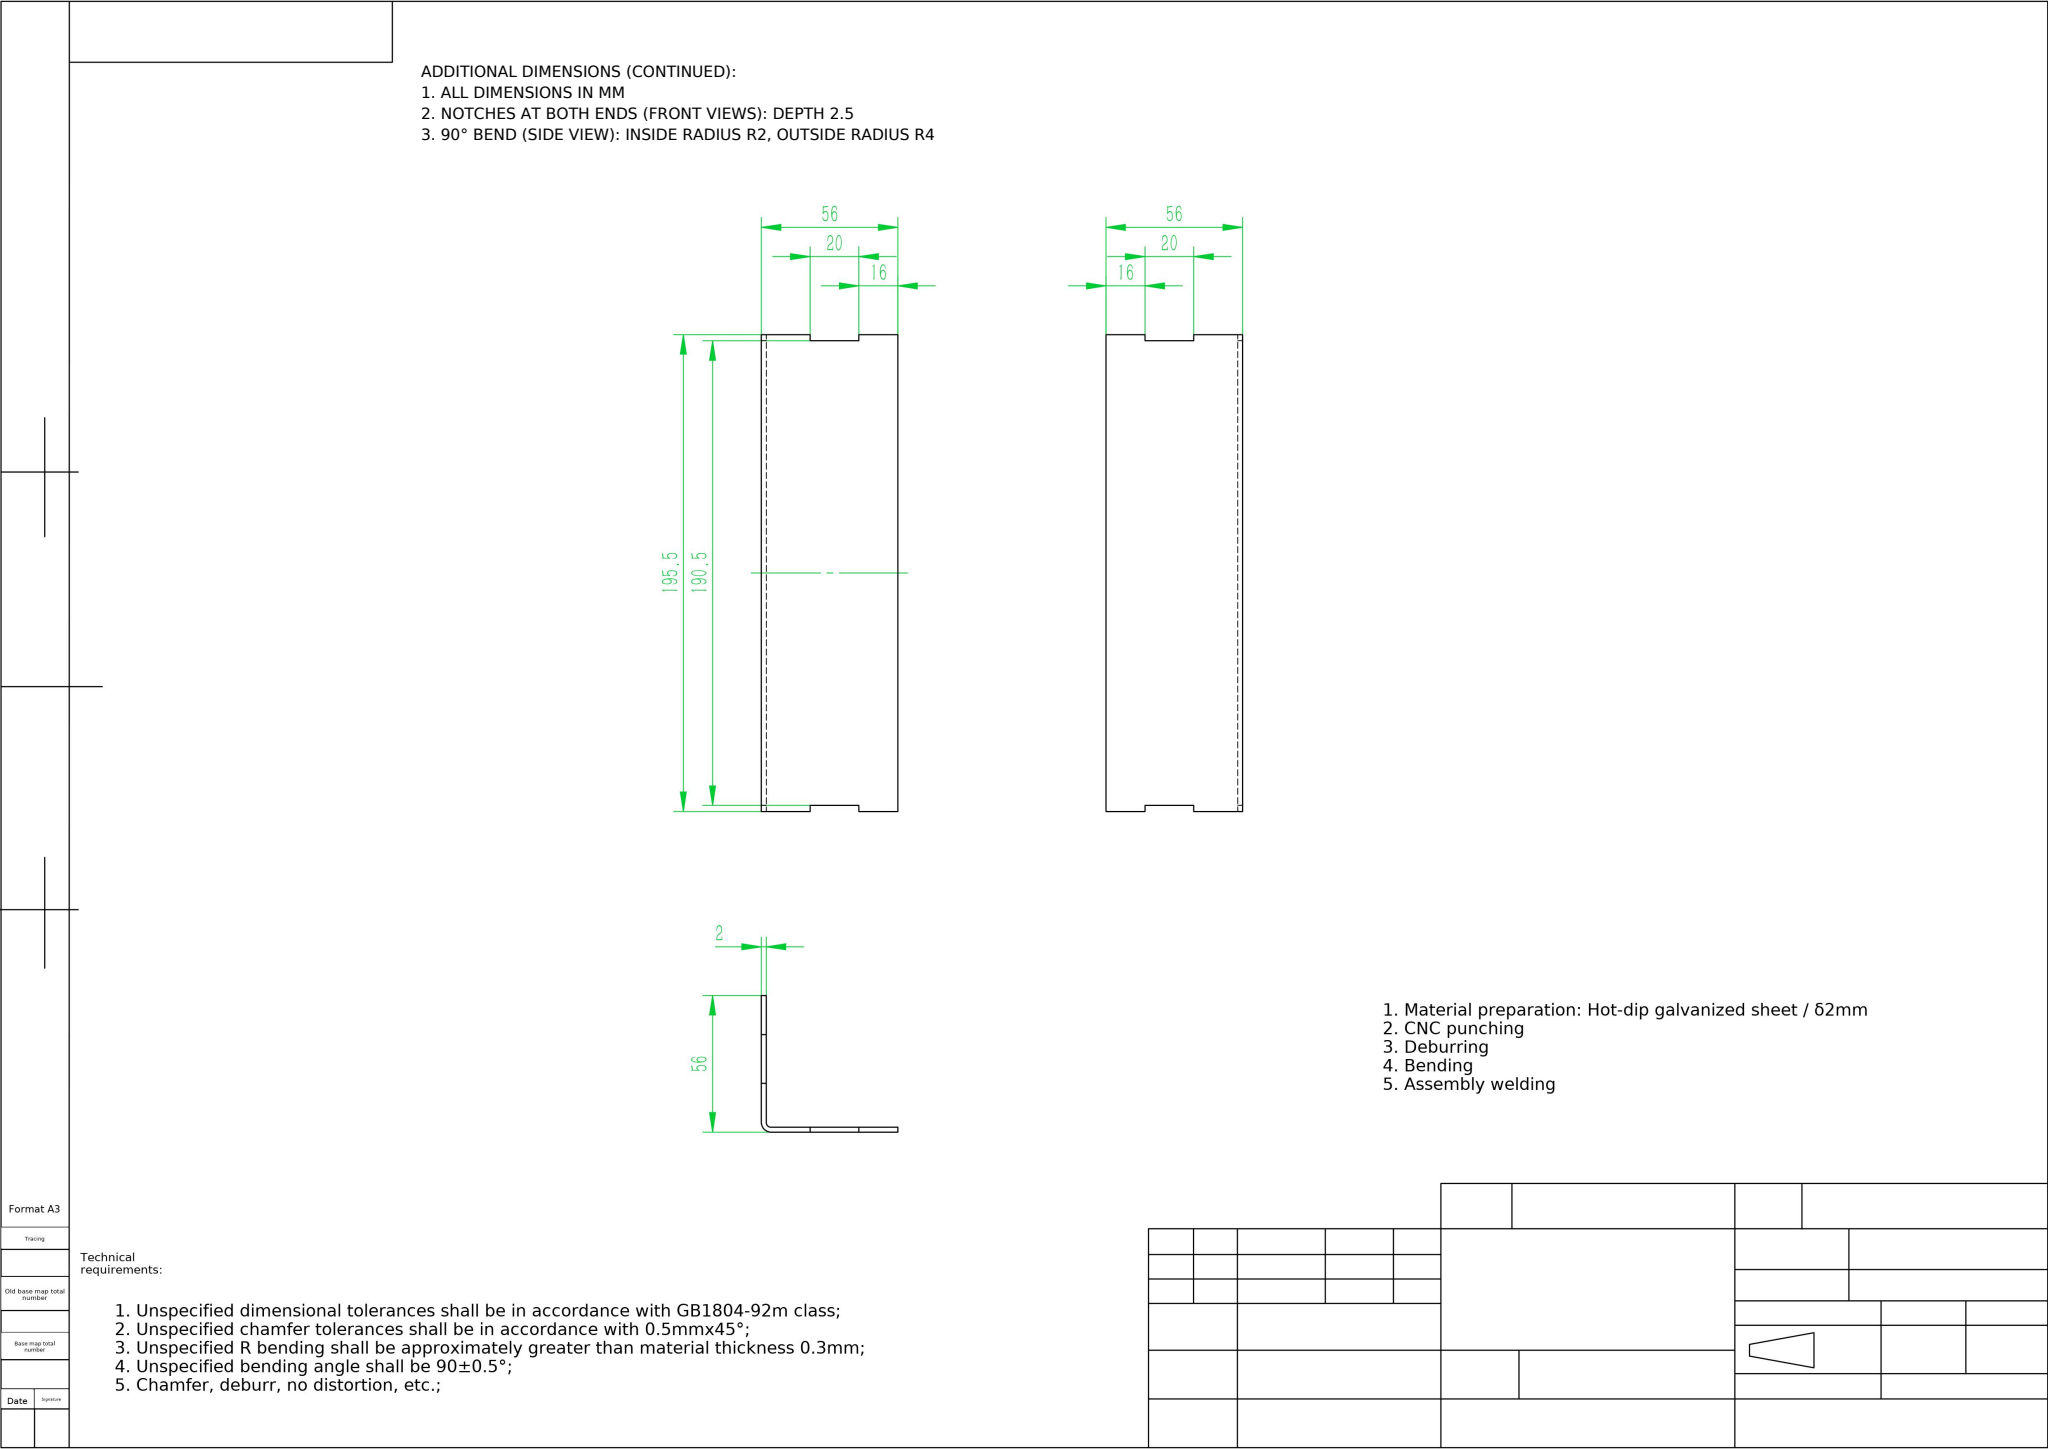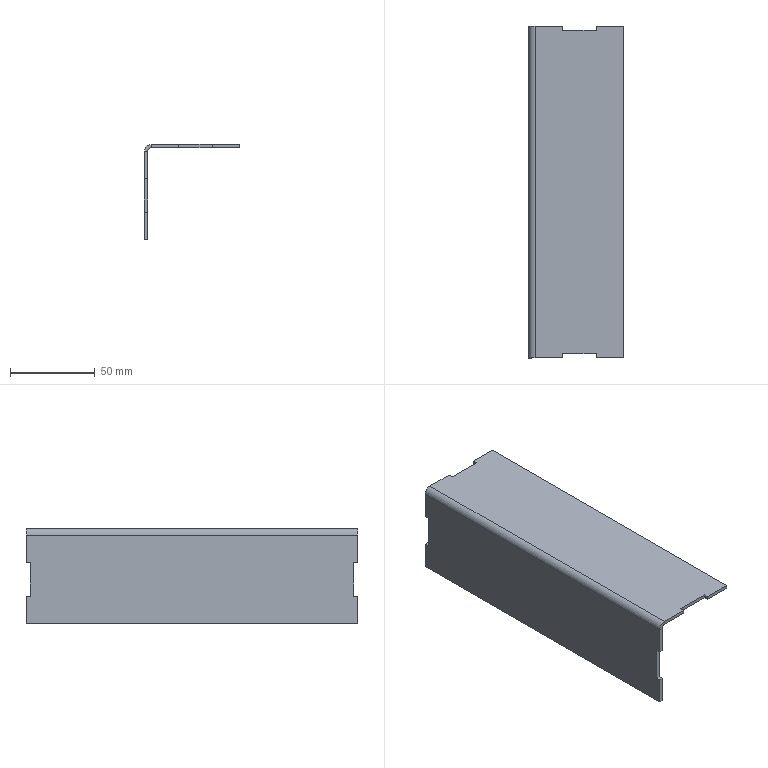Part | NX | mm | 1 solid | 30 faces | box 56 x 195.5 x 56 mm | volume 42107 mm3 | plane 28 | cylinder 2 | commonest cylinder face diameters 8 x1 4 x1
STEP:
#1=COLOUR_RGB('',0.7529,0.7529,0.7529);
#2=FILL_AREA_STYLE_COLOUR('',#1);
#3=FILL_AREA_STYLE('',(#2));
#4=SURFACE_STYLE_FILL_AREA(#3);
#5=SURFACE_SIDE_STYLE('',(#4));
#6=SURFACE_STYLE_USAGE(.BOTH.,#5);
#7=PRESENTATION_STYLE_ASSIGNMENT((#6));
#8=CARTESIAN_POINT('',(-28.,-97.75,-4.));
#9=VERTEX_POINT('',#8);
#10=CARTESIAN_POINT('',(-28.,-97.75,-20.));
#11=VERTEX_POINT('',#10);
#12=CARTESIAN_POINT('',(-28.,-97.75,-56.));
#13=DIRECTION('',(-0.,0.,-1.));
#14=VECTOR('',#13,1000.);
#15=LINE('',#12,#14);
#16=EDGE_CURVE('',#9,#11,#15,.T.);
#17=ORIENTED_EDGE('',*,*,#16,.T.);
#18=CARTESIAN_POINT('',(-26.,-97.75,-20.));
#19=VERTEX_POINT('',#18);
#20=CARTESIAN_POINT('',(-28.,-97.75,-20.));
#21=DIRECTION('',(1.,0.,-0.));
#22=VECTOR('',#21,1000.);
#23=LINE('',#20,#22);
#24=EDGE_CURVE('',#11,#19,#23,.T.);
#25=ORIENTED_EDGE('',*,*,#24,.T.);
#26=CARTESIAN_POINT('',(-26.,-97.75,-4.));
#27=VERTEX_POINT('',#26);
#28=CARTESIAN_POINT('',(-26.,-97.75,0.));
#29=DIRECTION('',(-0.,0.,-1.));
#30=VECTOR('',#29,1000.);
#31=LINE('',#28,#30);
#32=EDGE_CURVE('',#27,#19,#31,.T.);
#33=ORIENTED_EDGE('',*,*,#32,.F.);
#34=CARTESIAN_POINT('',(-28.,-97.75,-4.));
#35=DIRECTION('',(-1.,0.,0.));
#36=VECTOR('',#35,1000.);
#37=LINE('',#34,#36);
#38=EDGE_CURVE('',#27,#9,#37,.T.);
#39=ORIENTED_EDGE('',*,*,#38,.T.);
#40=EDGE_LOOP('',(#17,#25,#33,#39));
#41=FACE_OUTER_BOUND('',#40,.T.);
#42=CARTESIAN_POINT('',(-28.,-97.75,-56.));
#43=DIRECTION('',(0.,-1.,0.));
#44=DIRECTION('',(0.,0.,-1.));
#45=AXIS2_PLACEMENT_3D('',#42,#43,#44);
#46=PLANE('',#45);
#47=ADVANCED_FACE('',(#41),#46,.T.);
#48=CARTESIAN_POINT('',(-26.,-97.75,-40.));
#49=VERTEX_POINT('',#48);
#50=CARTESIAN_POINT('',(-26.,-97.75,-56.));
#51=VERTEX_POINT('',#50);
#52=CARTESIAN_POINT('',(-26.,-97.75,0.));
#53=DIRECTION('',(-0.,0.,-1.));
#54=VECTOR('',#53,1000.);
#55=LINE('',#52,#54);
#56=EDGE_CURVE('',#49,#51,#55,.T.);
#57=ORIENTED_EDGE('',*,*,#56,.F.);
#58=CARTESIAN_POINT('',(-28.,-97.75,-40.));
#59=VERTEX_POINT('',#58);
#60=CARTESIAN_POINT('',(-28.,-97.75,-40.));
#61=DIRECTION('',(-1.,0.,0.));
#62=VECTOR('',#61,1000.);
#63=LINE('',#60,#62);
#64=EDGE_CURVE('',#49,#59,#63,.T.);
#65=ORIENTED_EDGE('',*,*,#64,.T.);
#66=CARTESIAN_POINT('',(-28.,-97.75,-56.));
#67=VERTEX_POINT('',#66);
#68=CARTESIAN_POINT('',(-28.,-97.75,-56.));
#69=DIRECTION('',(-0.,0.,-1.));
#70=VECTOR('',#69,1000.);
#71=LINE('',#68,#70);
#72=EDGE_CURVE('',#59,#67,#71,.T.);
#73=ORIENTED_EDGE('',*,*,#72,.T.);
#74=CARTESIAN_POINT('',(-28.,-97.75,-56.));
#75=DIRECTION('',(1.,0.,-0.));
#76=VECTOR('',#75,1000.);
#77=LINE('',#74,#76);
#78=EDGE_CURVE('',#67,#51,#77,.T.);
#79=ORIENTED_EDGE('',*,*,#78,.T.);
#80=EDGE_LOOP('',(#57,#65,#73,#79));
#81=FACE_OUTER_BOUND('',#80,.T.);
#82=CARTESIAN_POINT('',(-28.,-97.75,-56.));
#83=DIRECTION('',(0.,-1.,0.));
#84=DIRECTION('',(0.,0.,-1.));
#85=AXIS2_PLACEMENT_3D('',#82,#83,#84);
#86=PLANE('',#85);
#87=ADVANCED_FACE('',(#81),#86,.T.);
#88=CARTESIAN_POINT('',(-28.,-95.25,-40.));
#89=VERTEX_POINT('',#88);
#90=CARTESIAN_POINT('',(-28.,-95.25,-20.));
#91=VERTEX_POINT('',#90);
#92=CARTESIAN_POINT('',(-28.,-95.25,-40.));
#93=DIRECTION('',(0.,0.,1.));
#94=VECTOR('',#93,1000.);
#95=LINE('',#92,#94);
#96=EDGE_CURVE('',#89,#91,#95,.T.);
#97=ORIENTED_EDGE('',*,*,#96,.T.);
#98=CARTESIAN_POINT('',(-28.,-100.25,-20.));
#99=DIRECTION('',(0.,-1.,0.));
#100=VECTOR('',#99,1000.);
#101=LINE('',#98,#100);
#102=EDGE_CURVE('',#91,#11,#101,.T.);
#103=ORIENTED_EDGE('',*,*,#102,.T.);
#104=ORIENTED_EDGE('',*,*,#16,.F.);
#105=CARTESIAN_POINT('',(-28.,97.75,-4.));
#106=VERTEX_POINT('',#105);
#107=CARTESIAN_POINT('',(-28.,0.,-4.));
#108=DIRECTION('',(0.,1.,0.));
#109=VECTOR('',#108,1000.);
#110=LINE('',#107,#109);
#111=EDGE_CURVE('',#9,#106,#110,.T.);
#112=ORIENTED_EDGE('',*,*,#111,.T.);
#113=CARTESIAN_POINT('',(-28.,97.75,-20.));
#114=VERTEX_POINT('',#113);
#115=CARTESIAN_POINT('',(-28.,97.75,-2.));
#116=DIRECTION('',(0.,0.,1.));
#117=VECTOR('',#116,1000.);
#118=LINE('',#115,#117);
#119=EDGE_CURVE('',#114,#106,#118,.T.);
#120=ORIENTED_EDGE('',*,*,#119,.F.);
#121=CARTESIAN_POINT('',(-28.,95.25,-20.));
#122=VERTEX_POINT('',#121);
#123=CARTESIAN_POINT('',(-28.,100.25,-20.));
#124=DIRECTION('',(0.,1.,0.));
#125=VECTOR('',#124,1000.);
#126=LINE('',#123,#125);
#127=EDGE_CURVE('',#122,#114,#126,.T.);
#128=ORIENTED_EDGE('',*,*,#127,.F.);
#129=CARTESIAN_POINT('',(-28.,95.25,-40.));
#130=VERTEX_POINT('',#129);
#131=CARTESIAN_POINT('',(-28.,95.25,-40.));
#132=DIRECTION('',(0.,0.,1.));
#133=VECTOR('',#132,1000.);
#134=LINE('',#131,#133);
#135=EDGE_CURVE('',#130,#122,#134,.T.);
#136=ORIENTED_EDGE('',*,*,#135,.F.);
#137=CARTESIAN_POINT('',(-28.,97.75,-40.));
#138=VERTEX_POINT('',#137);
#139=CARTESIAN_POINT('',(-28.,100.25,-40.));
#140=DIRECTION('',(0.,-1.,0.));
#141=VECTOR('',#140,1000.);
#142=LINE('',#139,#141);
#143=EDGE_CURVE('',#138,#130,#142,.T.);
#144=ORIENTED_EDGE('',*,*,#143,.F.);
#145=CARTESIAN_POINT('',(-28.,97.75,-56.));
#146=VERTEX_POINT('',#145);
#147=CARTESIAN_POINT('',(-28.,97.75,-2.));
#148=DIRECTION('',(0.,0.,1.));
#149=VECTOR('',#148,1000.);
#150=LINE('',#147,#149);
#151=EDGE_CURVE('',#146,#138,#150,.T.);
#152=ORIENTED_EDGE('',*,*,#151,.F.);
#153=CARTESIAN_POINT('',(-28.,97.75,-56.));
#154=DIRECTION('',(0.,1.,0.));
#155=VECTOR('',#154,1000.);
#156=LINE('',#153,#155);
#157=EDGE_CURVE('',#67,#146,#156,.T.);
#158=ORIENTED_EDGE('',*,*,#157,.F.);
#159=ORIENTED_EDGE('',*,*,#72,.F.);
#160=CARTESIAN_POINT('',(-28.,-100.25,-40.));
#161=DIRECTION('',(0.,1.,0.));
#162=VECTOR('',#161,1000.);
#163=LINE('',#160,#162);
#164=EDGE_CURVE('',#59,#89,#163,.T.);
#165=ORIENTED_EDGE('',*,*,#164,.T.);
#166=EDGE_LOOP('',(#97,#103,#104,#112,#120,#128,#136,#144,#152,#158,#159,#165));
#167=FACE_OUTER_BOUND('',#166,.T.);
#168=CARTESIAN_POINT('',(-28.,0.,0.));
#169=DIRECTION('',(-1.,0.,0.));
#170=DIRECTION('',(0.,0.,1.));
#171=AXIS2_PLACEMENT_3D('',#168,#169,#170);
#172=PLANE('',#171);
#173=ADVANCED_FACE('',(#167),#172,.T.);
#174=CARTESIAN_POINT('',(-26.,-95.25,-20.));
#175=VERTEX_POINT('',#174);
#176=CARTESIAN_POINT('',(-26.,-100.25,-20.));
#177=DIRECTION('',(0.,-1.,0.));
#178=VECTOR('',#177,1000.);
#179=LINE('',#176,#178);
#180=EDGE_CURVE('',#175,#19,#179,.T.);
#181=ORIENTED_EDGE('',*,*,#180,.F.);
#182=CARTESIAN_POINT('',(-26.,-95.25,-40.));
#183=VERTEX_POINT('',#182);
#184=CARTESIAN_POINT('',(-26.,-95.25,-40.));
#185=DIRECTION('',(0.,0.,1.));
#186=VECTOR('',#185,1000.);
#187=LINE('',#184,#186);
#188=EDGE_CURVE('',#183,#175,#187,.T.);
#189=ORIENTED_EDGE('',*,*,#188,.F.);
#190=CARTESIAN_POINT('',(-26.,0.,-40.));
#191=DIRECTION('',(0.,1.,0.));
#192=VECTOR('',#191,1000.);
#193=LINE('',#190,#192);
#194=EDGE_CURVE('',#49,#183,#193,.T.);
#195=ORIENTED_EDGE('',*,*,#194,.F.);
#196=ORIENTED_EDGE('',*,*,#56,.T.);
#197=CARTESIAN_POINT('',(-26.,97.75,-56.));
#198=VERTEX_POINT('',#197);
#199=CARTESIAN_POINT('',(-26.,0.,-56.));
#200=DIRECTION('',(0.,1.,0.));
#201=VECTOR('',#200,1000.);
#202=LINE('',#199,#201);
#203=EDGE_CURVE('',#51,#198,#202,.T.);
#204=ORIENTED_EDGE('',*,*,#203,.T.);
#205=CARTESIAN_POINT('',(-26.,97.75,-40.));
#206=VERTEX_POINT('',#205);
#207=CARTESIAN_POINT('',(-26.,97.75,0.));
#208=DIRECTION('',(0.,0.,1.));
#209=VECTOR('',#208,1000.);
#210=LINE('',#207,#209);
#211=EDGE_CURVE('',#198,#206,#210,.T.);
#212=ORIENTED_EDGE('',*,*,#211,.T.);
#213=CARTESIAN_POINT('',(-26.,95.25,-40.));
#214=VERTEX_POINT('',#213);
#215=CARTESIAN_POINT('',(-26.,0.,-40.));
#216=DIRECTION('',(0.,-1.,0.));
#217=VECTOR('',#216,1000.);
#218=LINE('',#215,#217);
#219=EDGE_CURVE('',#206,#214,#218,.T.);
#220=ORIENTED_EDGE('',*,*,#219,.T.);
#221=CARTESIAN_POINT('',(-26.,95.25,-20.));
#222=VERTEX_POINT('',#221);
#223=CARTESIAN_POINT('',(-26.,95.25,-40.));
#224=DIRECTION('',(0.,0.,1.));
#225=VECTOR('',#224,1000.);
#226=LINE('',#223,#225);
#227=EDGE_CURVE('',#214,#222,#226,.T.);
#228=ORIENTED_EDGE('',*,*,#227,.T.);
#229=CARTESIAN_POINT('',(-26.,97.75,-20.));
#230=VERTEX_POINT('',#229);
#231=CARTESIAN_POINT('',(-26.,100.25,-20.));
#232=DIRECTION('',(0.,1.,0.));
#233=VECTOR('',#232,1000.);
#234=LINE('',#231,#233);
#235=EDGE_CURVE('',#222,#230,#234,.T.);
#236=ORIENTED_EDGE('',*,*,#235,.T.);
#237=CARTESIAN_POINT('',(-26.,97.75,-4.));
#238=VERTEX_POINT('',#237);
#239=CARTESIAN_POINT('',(-26.,97.75,0.));
#240=DIRECTION('',(0.,0.,1.));
#241=VECTOR('',#240,1000.);
#242=LINE('',#239,#241);
#243=EDGE_CURVE('',#230,#238,#242,.T.);
#244=ORIENTED_EDGE('',*,*,#243,.T.);
#245=CARTESIAN_POINT('',(-26.,-97.75,-4.));
#246=DIRECTION('',(0.,1.,0.));
#247=VECTOR('',#246,1000.);
#248=LINE('',#245,#247);
#249=EDGE_CURVE('',#27,#238,#248,.T.);
#250=ORIENTED_EDGE('',*,*,#249,.F.);
#251=ORIENTED_EDGE('',*,*,#32,.T.);
#252=EDGE_LOOP('',(#181,#189,#195,#196,#204,#212,#220,#228,#236,#244,#250,#251));
#253=FACE_OUTER_BOUND('',#252,.T.);
#254=CARTESIAN_POINT('',(-26.,0.,0.));
#255=DIRECTION('',(-1.,0.,0.));
#256=DIRECTION('',(0.,0.,1.));
#257=AXIS2_PLACEMENT_3D('',#254,#255,#256);
#258=PLANE('',#257);
#259=ADVANCED_FACE('',(#253),#258,.F.);
#260=CARTESIAN_POINT('',(12.,-97.75,-2.));
#261=VERTEX_POINT('',#260);
#262=CARTESIAN_POINT('',(28.,-97.75,-2.));
#263=VERTEX_POINT('',#262);
#264=CARTESIAN_POINT('',(-28.,-97.75,-2.));
#265=DIRECTION('',(1.,0.,0.));
#266=VECTOR('',#265,1000.);
#267=LINE('',#264,#266);
#268=EDGE_CURVE('',#261,#263,#267,.T.);
#269=ORIENTED_EDGE('',*,*,#268,.F.);
#270=CARTESIAN_POINT('',(12.,-95.25,-2.));
#271=VERTEX_POINT('',#270);
#272=CARTESIAN_POINT('',(12.,-100.25,-2.));
#273=DIRECTION('',(0.,-1.,0.));
#274=VECTOR('',#273,1000.);
#275=LINE('',#272,#274);
#276=EDGE_CURVE('',#271,#261,#275,.T.);
#277=ORIENTED_EDGE('',*,*,#276,.F.);
#278=CARTESIAN_POINT('',(-8.,-95.25,-2.));
#279=VERTEX_POINT('',#278);
#280=CARTESIAN_POINT('',(-8.,-95.25,-2.));
#281=DIRECTION('',(1.,0.,0.));
#282=VECTOR('',#281,1000.);
#283=LINE('',#280,#282);
#284=EDGE_CURVE('',#279,#271,#283,.T.);
#285=ORIENTED_EDGE('',*,*,#284,.F.);
#286=CARTESIAN_POINT('',(-8.,-97.75,-2.));
#287=VERTEX_POINT('',#286);
#288=CARTESIAN_POINT('',(-8.,-100.25,-2.));
#289=DIRECTION('',(0.,1.,0.));
#290=VECTOR('',#289,1000.);
#291=LINE('',#288,#290);
#292=EDGE_CURVE('',#287,#279,#291,.T.);
#293=ORIENTED_EDGE('',*,*,#292,.F.);
#294=CARTESIAN_POINT('',(-24.,-97.75,-2.));
#295=VERTEX_POINT('',#294);
#296=CARTESIAN_POINT('',(-28.,-97.75,-2.));
#297=DIRECTION('',(1.,0.,0.));
#298=VECTOR('',#297,1000.);
#299=LINE('',#296,#298);
#300=EDGE_CURVE('',#295,#287,#299,.T.);
#301=ORIENTED_EDGE('',*,*,#300,.F.);
#302=CARTESIAN_POINT('',(-24.,97.75,-2.));
#303=VERTEX_POINT('',#302);
#304=CARTESIAN_POINT('',(-24.,97.75,-2.));
#305=DIRECTION('',(0.,-1.,0.));
#306=VECTOR('',#305,1000.);
#307=LINE('',#304,#306);
#308=EDGE_CURVE('',#303,#295,#307,.T.);
#309=ORIENTED_EDGE('',*,*,#308,.F.);
#310=CARTESIAN_POINT('',(-8.,97.75,-2.));
#311=VERTEX_POINT('',#310);
#312=CARTESIAN_POINT('',(-28.,97.75,-2.));
#313=DIRECTION('',(-1.,0.,0.));
#314=VECTOR('',#313,1000.);
#315=LINE('',#312,#314);
#316=EDGE_CURVE('',#311,#303,#315,.T.);
#317=ORIENTED_EDGE('',*,*,#316,.F.);
#318=CARTESIAN_POINT('',(-8.,95.25,-2.));
#319=VERTEX_POINT('',#318);
#320=CARTESIAN_POINT('',(-8.,100.25,-2.));
#321=DIRECTION('',(0.,-1.,0.));
#322=VECTOR('',#321,1000.);
#323=LINE('',#320,#322);
#324=EDGE_CURVE('',#311,#319,#323,.T.);
#325=ORIENTED_EDGE('',*,*,#324,.T.);
#326=CARTESIAN_POINT('',(12.,95.25,-2.));
#327=VERTEX_POINT('',#326);
#328=CARTESIAN_POINT('',(-8.,95.25,-2.));
#329=DIRECTION('',(1.,0.,0.));
#330=VECTOR('',#329,1000.);
#331=LINE('',#328,#330);
#332=EDGE_CURVE('',#319,#327,#331,.T.);
#333=ORIENTED_EDGE('',*,*,#332,.T.);
#334=CARTESIAN_POINT('',(12.,97.75,-2.));
#335=VERTEX_POINT('',#334);
#336=CARTESIAN_POINT('',(12.,100.25,-2.));
#337=DIRECTION('',(0.,1.,0.));
#338=VECTOR('',#337,1000.);
#339=LINE('',#336,#338);
#340=EDGE_CURVE('',#327,#335,#339,.T.);
#341=ORIENTED_EDGE('',*,*,#340,.T.);
#342=CARTESIAN_POINT('',(28.,97.75,-2.));
#343=VERTEX_POINT('',#342);
#344=CARTESIAN_POINT('',(-28.,97.75,-2.));
#345=DIRECTION('',(-1.,0.,0.));
#346=VECTOR('',#345,1000.);
#347=LINE('',#344,#346);
#348=EDGE_CURVE('',#343,#335,#347,.T.);
#349=ORIENTED_EDGE('',*,*,#348,.F.);
#350=CARTESIAN_POINT('',(28.,-97.75,-2.));
#351=DIRECTION('',(0.,1.,0.));
#352=VECTOR('',#351,1000.);
#353=LINE('',#350,#352);
#354=EDGE_CURVE('',#263,#343,#353,.T.);
#355=ORIENTED_EDGE('',*,*,#354,.F.);
#356=EDGE_LOOP('',(#269,#277,#285,#293,#301,#309,#317,#325,#333,#341,#349,#355));
#357=FACE_OUTER_BOUND('',#356,.T.);
#358=CARTESIAN_POINT('',(0.,0.,-2.));
#359=DIRECTION('',(0.,0.,-1.));
#360=DIRECTION('',(-1.,0.,0.));
#361=AXIS2_PLACEMENT_3D('',#358,#359,#360);
#362=PLANE('',#361);
#363=ADVANCED_FACE('',(#357),#362,.T.);
#364=CARTESIAN_POINT('',(12.,-95.25,0.));
#365=VERTEX_POINT('',#364);
#366=CARTESIAN_POINT('',(12.,-97.75,0.));
#367=VERTEX_POINT('',#366);
#368=CARTESIAN_POINT('',(12.,-100.25,0.));
#369=DIRECTION('',(0.,-1.,0.));
#370=VECTOR('',#369,1000.);
#371=LINE('',#368,#370);
#372=EDGE_CURVE('',#365,#367,#371,.T.);
#373=ORIENTED_EDGE('',*,*,#372,.T.);
#374=CARTESIAN_POINT('',(28.,-97.75,0.));
#375=VERTEX_POINT('',#374);
#376=CARTESIAN_POINT('',(-28.,-97.75,0.));
#377=DIRECTION('',(1.,0.,0.));
#378=VECTOR('',#377,1000.);
#379=LINE('',#376,#378);
#380=EDGE_CURVE('',#367,#375,#379,.T.);
#381=ORIENTED_EDGE('',*,*,#380,.T.);
#382=CARTESIAN_POINT('',(28.,97.75,0.));
#383=VERTEX_POINT('',#382);
#384=CARTESIAN_POINT('',(28.,-97.75,0.));
#385=DIRECTION('',(0.,1.,0.));
#386=VECTOR('',#385,1000.);
#387=LINE('',#384,#386);
#388=EDGE_CURVE('',#375,#383,#387,.T.);
#389=ORIENTED_EDGE('',*,*,#388,.T.);
#390=CARTESIAN_POINT('',(12.,97.75,0.));
#391=VERTEX_POINT('',#390);
#392=CARTESIAN_POINT('',(-28.,97.75,0.));
#393=DIRECTION('',(-1.,0.,0.));
#394=VECTOR('',#393,1000.);
#395=LINE('',#392,#394);
#396=EDGE_CURVE('',#383,#391,#395,.T.);
#397=ORIENTED_EDGE('',*,*,#396,.T.);
#398=CARTESIAN_POINT('',(12.,95.25,0.));
#399=VERTEX_POINT('',#398);
#400=CARTESIAN_POINT('',(12.,100.25,0.));
#401=DIRECTION('',(0.,1.,0.));
#402=VECTOR('',#401,1000.);
#403=LINE('',#400,#402);
#404=EDGE_CURVE('',#399,#391,#403,.T.);
#405=ORIENTED_EDGE('',*,*,#404,.F.);
#406=CARTESIAN_POINT('',(-8.,95.25,0.));
#407=VERTEX_POINT('',#406);
#408=CARTESIAN_POINT('',(-8.,95.25,0.));
#409=DIRECTION('',(1.,0.,0.));
#410=VECTOR('',#409,1000.);
#411=LINE('',#408,#410);
#412=EDGE_CURVE('',#407,#399,#411,.T.);
#413=ORIENTED_EDGE('',*,*,#412,.F.);
#414=CARTESIAN_POINT('',(-8.,97.75,0.));
#415=VERTEX_POINT('',#414);
#416=CARTESIAN_POINT('',(-8.,0.,0.));
#417=DIRECTION('',(0.,1.,0.));
#418=VECTOR('',#417,1000.);
#419=LINE('',#416,#418);
#420=EDGE_CURVE('',#407,#415,#419,.T.);
#421=ORIENTED_EDGE('',*,*,#420,.T.);
#422=CARTESIAN_POINT('',(-24.,97.75,0.));
#423=VERTEX_POINT('',#422);
#424=CARTESIAN_POINT('',(-28.,97.75,0.));
#425=DIRECTION('',(-1.,0.,0.));
#426=VECTOR('',#425,1000.);
#427=LINE('',#424,#426);
#428=EDGE_CURVE('',#415,#423,#427,.T.);
#429=ORIENTED_EDGE('',*,*,#428,.T.);
#430=CARTESIAN_POINT('',(-24.,-97.75,0.));
#431=VERTEX_POINT('',#430);
#432=CARTESIAN_POINT('',(-24.,97.75,0.));
#433=DIRECTION('',(0.,-1.,0.));
#434=VECTOR('',#433,1000.);
#435=LINE('',#432,#434);
#436=EDGE_CURVE('',#423,#431,#435,.T.);
#437=ORIENTED_EDGE('',*,*,#436,.T.);
#438=CARTESIAN_POINT('',(-8.,-97.75,0.));
#439=VERTEX_POINT('',#438);
#440=CARTESIAN_POINT('',(-28.,-97.75,0.));
#441=DIRECTION('',(1.,0.,0.));
#442=VECTOR('',#441,1000.);
#443=LINE('',#440,#442);
#444=EDGE_CURVE('',#431,#439,#443,.T.);
#445=ORIENTED_EDGE('',*,*,#444,.T.);
#446=CARTESIAN_POINT('',(-8.,-95.25,0.));
#447=VERTEX_POINT('',#446);
#448=CARTESIAN_POINT('',(-8.,-100.25,0.));
#449=DIRECTION('',(0.,1.,0.));
#450=VECTOR('',#449,1000.);
#451=LINE('',#448,#450);
#452=EDGE_CURVE('',#439,#447,#451,.T.);
#453=ORIENTED_EDGE('',*,*,#452,.T.);
#454=CARTESIAN_POINT('',(-8.,-95.25,0.));
#455=DIRECTION('',(1.,0.,0.));
#456=VECTOR('',#455,1000.);
#457=LINE('',#454,#456);
#458=EDGE_CURVE('',#447,#365,#457,.T.);
#459=ORIENTED_EDGE('',*,*,#458,.T.);
#460=EDGE_LOOP('',(#373,#381,#389,#397,#405,#413,#421,#429,#437,#445,#453,#459));
#461=FACE_OUTER_BOUND('',#460,.T.);
#462=CARTESIAN_POINT('',(0.,0.,0.));
#463=DIRECTION('',(0.,0.,-1.));
#464=DIRECTION('',(-1.,0.,0.));
#465=AXIS2_PLACEMENT_3D('',#462,#463,#464);
#466=PLANE('',#465);
#467=ADVANCED_FACE('',(#461),#466,.F.);
#468=ORIENTED_EDGE('',*,*,#380,.F.);
#469=CARTESIAN_POINT('',(12.,-97.75,-2.));
#470=DIRECTION('',(0.,0.,-1.));
#471=VECTOR('',#470,1000.);
#472=LINE('',#469,#471);
#473=EDGE_CURVE('',#367,#261,#472,.T.);
#474=ORIENTED_EDGE('',*,*,#473,.T.);
#475=ORIENTED_EDGE('',*,*,#268,.T.);
#476=CARTESIAN_POINT('',(28.,-97.75,-2.));
#477=DIRECTION('',(0.,0.,1.));
#478=VECTOR('',#477,1000.);
#479=LINE('',#476,#478);
#480=EDGE_CURVE('',#263,#375,#479,.T.);
#481=ORIENTED_EDGE('',*,*,#480,.T.);
#482=EDGE_LOOP('',(#468,#474,#475,#481));
#483=FACE_OUTER_BOUND('',#482,.T.);
#484=CARTESIAN_POINT('',(-28.,-97.75,-2.));
#485=DIRECTION('',(0.,-1.,0.));
#486=DIRECTION('',(0.,0.,-1.));
#487=AXIS2_PLACEMENT_3D('',#484,#485,#486);
#488=PLANE('',#487);
#489=ADVANCED_FACE('',(#483),#488,.T.);
#490=ORIENTED_EDGE('',*,*,#300,.T.);
#491=CARTESIAN_POINT('',(-8.,-97.75,-2.));
#492=DIRECTION('',(0.,0.,1.));
#493=VECTOR('',#492,1000.);
#494=LINE('',#491,#493);
#495=EDGE_CURVE('',#287,#439,#494,.T.);
#496=ORIENTED_EDGE('',*,*,#495,.T.);
#497=ORIENTED_EDGE('',*,*,#444,.F.);
#498=CARTESIAN_POINT('',(-24.,-97.75,-2.));
#499=DIRECTION('',(0.,0.,1.));
#500=VECTOR('',#499,1000.);
#501=LINE('',#498,#500);
#502=EDGE_CURVE('',#295,#431,#501,.T.);
#503=ORIENTED_EDGE('',*,*,#502,.F.);
#504=EDGE_LOOP('',(#490,#496,#497,#503));
#505=FACE_OUTER_BOUND('',#504,.T.);
#506=CARTESIAN_POINT('',(-28.,-97.75,-2.));
#507=DIRECTION('',(0.,-1.,0.));
#508=DIRECTION('',(0.,0.,-1.));
#509=AXIS2_PLACEMENT_3D('',#506,#507,#508);
#510=PLANE('',#509);
#511=ADVANCED_FACE('',(#505),#510,.T.);
#512=CARTESIAN_POINT('',(-28.,97.75,-20.));
#513=DIRECTION('',(1.,0.,-0.));
#514=VECTOR('',#513,1000.);
#515=LINE('',#512,#514);
#516=EDGE_CURVE('',#114,#230,#515,.T.);
#517=ORIENTED_EDGE('',*,*,#516,.F.);
#518=ORIENTED_EDGE('',*,*,#119,.T.);
#519=CARTESIAN_POINT('',(-26.,97.75,-4.));
#520=DIRECTION('',(-1.,0.,0.));
#521=VECTOR('',#520,1000.);
#522=LINE('',#519,#521);
#523=EDGE_CURVE('',#238,#106,#522,.T.);
#524=ORIENTED_EDGE('',*,*,#523,.F.);
#525=ORIENTED_EDGE('',*,*,#243,.F.);
#526=EDGE_LOOP('',(#517,#518,#524,#525));
#527=FACE_OUTER_BOUND('',#526,.T.);
#528=CARTESIAN_POINT('',(-28.,97.75,-2.));
#529=DIRECTION('',(0.,1.,0.));
#530=DIRECTION('',(0.,0.,1.));
#531=AXIS2_PLACEMENT_3D('',#528,#529,#530);
#532=PLANE('',#531);
#533=ADVANCED_FACE('',(#527),#532,.T.);
#534=CARTESIAN_POINT('',(12.,97.75,-2.));
#535=DIRECTION('',(0.,0.,-1.));
#536=VECTOR('',#535,1000.);
#537=LINE('',#534,#536);
#538=EDGE_CURVE('',#391,#335,#537,.T.);
#539=ORIENTED_EDGE('',*,*,#538,.F.);
#540=ORIENTED_EDGE('',*,*,#396,.F.);
#541=CARTESIAN_POINT('',(28.,97.75,-2.));
#542=DIRECTION('',(0.,0.,1.));
#543=VECTOR('',#542,1000.);
#544=LINE('',#541,#543);
#545=EDGE_CURVE('',#343,#383,#544,.T.);
#546=ORIENTED_EDGE('',*,*,#545,.F.);
#547=ORIENTED_EDGE('',*,*,#348,.T.);
#548=EDGE_LOOP('',(#539,#540,#546,#547));
#549=FACE_OUTER_BOUND('',#548,.T.);
#550=CARTESIAN_POINT('',(-28.,97.75,-2.));
#551=DIRECTION('',(0.,1.,0.));
#552=DIRECTION('',(0.,0.,1.));
#553=AXIS2_PLACEMENT_3D('',#550,#551,#552);
#554=PLANE('',#553);
#555=ADVANCED_FACE('',(#549),#554,.T.);
#556=CARTESIAN_POINT('',(-8.,97.75,-2.));
#557=DIRECTION('',(0.,0.,1.));
#558=VECTOR('',#557,1000.);
#559=LINE('',#556,#558);
#560=EDGE_CURVE('',#311,#415,#559,.T.);
#561=ORIENTED_EDGE('',*,*,#560,.F.);
#562=ORIENTED_EDGE('',*,*,#316,.T.);
#563=CARTESIAN_POINT('',(-24.,97.75,-2.));
#564=DIRECTION('',(0.,0.,1.));
#565=VECTOR('',#564,1000.);
#566=LINE('',#563,#565);
#567=EDGE_CURVE('',#303,#423,#566,.T.);
#568=ORIENTED_EDGE('',*,*,#567,.T.);
#569=ORIENTED_EDGE('',*,*,#428,.F.);
#570=EDGE_LOOP('',(#561,#562,#568,#569));
#571=FACE_OUTER_BOUND('',#570,.T.);
#572=CARTESIAN_POINT('',(-28.,97.75,-2.));
#573=DIRECTION('',(0.,1.,0.));
#574=DIRECTION('',(0.,0.,1.));
#575=AXIS2_PLACEMENT_3D('',#572,#573,#574);
#576=PLANE('',#575);
#577=ADVANCED_FACE('',(#571),#576,.T.);
#578=ORIENTED_EDGE('',*,*,#388,.F.);
#579=ORIENTED_EDGE('',*,*,#480,.F.);
#580=ORIENTED_EDGE('',*,*,#354,.T.);
#581=ORIENTED_EDGE('',*,*,#545,.T.);
#582=EDGE_LOOP('',(#578,#579,#580,#581));
#583=FACE_OUTER_BOUND('',#582,.T.);
#584=CARTESIAN_POINT('',(28.,-97.75,-2.));
#585=DIRECTION('',(1.,0.,0.));
#586=DIRECTION('',(0.,0.,-1.));
#587=AXIS2_PLACEMENT_3D('',#584,#585,#586);
#588=PLANE('',#587);
#589=ADVANCED_FACE('',(#583),#588,.T.);
#590=ORIENTED_EDGE('',*,*,#38,.F.);
#591=CARTESIAN_POINT('',(-24.,-97.75,-4.));
#592=DIRECTION('',(0.,-1.,0.));
#593=DIRECTION('',(0.,0.,1.));
#594=AXIS2_PLACEMENT_3D('',#591,#592,#593);
#595=CIRCLE('',#594,2.);
#596=EDGE_CURVE('',#295,#27,#595,.T.);
#597=ORIENTED_EDGE('',*,*,#596,.F.);
#598=ORIENTED_EDGE('',*,*,#502,.T.);
#599=CARTESIAN_POINT('',(-24.,-97.75,-4.));
#600=DIRECTION('',(0.,-1.,0.));
#601=DIRECTION('',(0.,0.,1.));
#602=AXIS2_PLACEMENT_3D('',#599,#600,#601);
#603=CIRCLE('',#602,4.);
#604=EDGE_CURVE('',#431,#9,#603,.T.);
#605=ORIENTED_EDGE('',*,*,#604,.T.);
#606=EDGE_LOOP('',(#590,#597,#598,#605));
#607=FACE_OUTER_BOUND('',#606,.T.);
#608=CARTESIAN_POINT('',(-24.,-97.75,-4.));
#609=DIRECTION('',(0.,-1.,0.));
#610=DIRECTION('',(0.,0.,-1.));
#611=AXIS2_PLACEMENT_3D('',#608,#609,#610);
#612=PLANE('',#611);
#613=ADVANCED_FACE('',(#607),#612,.T.);
#614=CARTESIAN_POINT('',(-24.,97.75,-4.));
#615=DIRECTION('',(0.,1.,0.));
#616=DIRECTION('',(0.,0.,1.));
#617=AXIS2_PLACEMENT_3D('',#614,#615,#616);
#618=CIRCLE('',#617,2.);
#619=EDGE_CURVE('',#238,#303,#618,.T.);
#620=ORIENTED_EDGE('',*,*,#619,.F.);
#621=ORIENTED_EDGE('',*,*,#523,.T.);
#622=CARTESIAN_POINT('',(-24.,97.75,-4.));
#623=DIRECTION('',(0.,1.,0.));
#624=DIRECTION('',(0.,0.,1.));
#625=AXIS2_PLACEMENT_3D('',#622,#623,#624);
#626=CIRCLE('',#625,4.);
#627=EDGE_CURVE('',#106,#423,#626,.T.);
#628=ORIENTED_EDGE('',*,*,#627,.T.);
#629=ORIENTED_EDGE('',*,*,#567,.F.);
#630=EDGE_LOOP('',(#620,#621,#628,#629));
#631=FACE_OUTER_BOUND('',#630,.T.);
#632=CARTESIAN_POINT('',(-24.,97.75,-4.));
#633=DIRECTION('',(0.,-1.,0.));
#634=DIRECTION('',(0.,0.,-1.));
#635=AXIS2_PLACEMENT_3D('',#632,#633,#634);
#636=PLANE('',#635);
#637=ADVANCED_FACE('',(#631),#636,.F.);
#638=ORIENTED_EDGE('',*,*,#436,.F.);
#639=ORIENTED_EDGE('',*,*,#627,.F.);
#640=ORIENTED_EDGE('',*,*,#111,.F.);
#641=ORIENTED_EDGE('',*,*,#604,.F.);
#642=EDGE_LOOP('',(#638,#639,#640,#641));
#643=FACE_OUTER_BOUND('',#642,.T.);
#644=CARTESIAN_POINT('',(-24.,97.75,-4.));
#645=DIRECTION('',(0.,1.,0.));
#646=DIRECTION('',(-1.,0.,0.));
#647=AXIS2_PLACEMENT_3D('',#644,#645,#646);
#648=CYLINDRICAL_SURFACE('',#647,4.);
#649=ADVANCED_FACE('',(#643),#648,.T.);
#650=ORIENTED_EDGE('',*,*,#308,.T.);
#651=ORIENTED_EDGE('',*,*,#596,.T.);
#652=ORIENTED_EDGE('',*,*,#249,.T.);
#653=ORIENTED_EDGE('',*,*,#619,.T.);
#654=EDGE_LOOP('',(#650,#651,#652,#653));
#655=FACE_OUTER_BOUND('',#654,.T.);
#656=CARTESIAN_POINT('',(-24.,97.75,-4.));
#657=DIRECTION('',(0.,1.,0.));
#658=DIRECTION('',(-1.,0.,0.));
#659=AXIS2_PLACEMENT_3D('',#656,#657,#658);
#660=CYLINDRICAL_SURFACE('',#659,2.);
#661=ADVANCED_FACE('',(#655),#660,.F.);
#662=CARTESIAN_POINT('',(-28.,97.75,-40.));
#663=DIRECTION('',(-1.,0.,0.));
#664=VECTOR('',#663,1000.);
#665=LINE('',#662,#664);
#666=EDGE_CURVE('',#206,#138,#665,.T.);
#667=ORIENTED_EDGE('',*,*,#666,.F.);
#668=ORIENTED_EDGE('',*,*,#211,.F.);
#669=CARTESIAN_POINT('',(-28.,97.75,-56.));
#670=DIRECTION('',(1.,0.,-0.));
#671=VECTOR('',#670,1000.);
#672=LINE('',#669,#671);
#673=EDGE_CURVE('',#146,#198,#672,.T.);
#674=ORIENTED_EDGE('',*,*,#673,.F.);
#675=ORIENTED_EDGE('',*,*,#151,.T.);
#676=EDGE_LOOP('',(#667,#668,#674,#675));
#677=FACE_OUTER_BOUND('',#676,.T.);
#678=CARTESIAN_POINT('',(-28.,97.75,-2.));
#679=DIRECTION('',(0.,1.,0.));
#680=DIRECTION('',(0.,0.,1.));
#681=AXIS2_PLACEMENT_3D('',#678,#679,#680);
#682=PLANE('',#681);
#683=ADVANCED_FACE('',(#677),#682,.T.);
#684=ORIENTED_EDGE('',*,*,#203,.F.);
#685=ORIENTED_EDGE('',*,*,#78,.F.);
#686=ORIENTED_EDGE('',*,*,#157,.T.);
#687=ORIENTED_EDGE('',*,*,#673,.T.);
#688=EDGE_LOOP('',(#684,#685,#686,#687));
#689=FACE_OUTER_BOUND('',#688,.T.);
#690=CARTESIAN_POINT('',(-28.,97.75,-56.));
#691=DIRECTION('',(-0.,0.,-1.));
#692=DIRECTION('',(-1.,0.,0.));
#693=AXIS2_PLACEMENT_3D('',#690,#691,#692);
#694=PLANE('',#693);
#695=ADVANCED_FACE('',(#689),#694,.T.);
#696=ORIENTED_EDGE('',*,*,#538,.T.);
#697=ORIENTED_EDGE('',*,*,#340,.F.);
#698=CARTESIAN_POINT('',(12.,95.25,-2.));
#699=DIRECTION('',(0.,0.,1.));
#700=VECTOR('',#699,1000.);
#701=LINE('',#698,#700);
#702=EDGE_CURVE('',#327,#399,#701,.T.);
#703=ORIENTED_EDGE('',*,*,#702,.T.);
#704=ORIENTED_EDGE('',*,*,#404,.T.);
#705=EDGE_LOOP('',(#696,#697,#703,#704));
#706=FACE_OUTER_BOUND('',#705,.T.);
#707=CARTESIAN_POINT('',(12.,100.25,-2.));
#708=DIRECTION('',(1.,0.,0.));
#709=DIRECTION('',(0.,0.,-1.));
#710=AXIS2_PLACEMENT_3D('',#707,#708,#709);
#711=PLANE('',#710);
#712=ADVANCED_FACE('',(#706),#711,.F.);
#713=ORIENTED_EDGE('',*,*,#412,.T.);
#714=ORIENTED_EDGE('',*,*,#702,.F.);
#715=ORIENTED_EDGE('',*,*,#332,.F.);
#716=CARTESIAN_POINT('',(-8.,95.25,-2.));
#717=DIRECTION('',(0.,0.,1.));
#718=VECTOR('',#717,1000.);
#719=LINE('',#716,#718);
#720=EDGE_CURVE('',#319,#407,#719,.T.);
#721=ORIENTED_EDGE('',*,*,#720,.T.);
#722=EDGE_LOOP('',(#713,#714,#715,#721));
#723=FACE_OUTER_BOUND('',#722,.T.);
#724=CARTESIAN_POINT('',(-8.,95.25,-2.));
#725=DIRECTION('',(0.,-1.,0.));
#726=DIRECTION('',(0.,0.,-1.));
#727=AXIS2_PLACEMENT_3D('',#724,#725,#726);
#728=PLANE('',#727);
#729=ADVANCED_FACE('',(#723),#728,.F.);
#730=ORIENTED_EDGE('',*,*,#560,.T.);
#731=ORIENTED_EDGE('',*,*,#420,.F.);
#732=ORIENTED_EDGE('',*,*,#720,.F.);
#733=ORIENTED_EDGE('',*,*,#324,.F.);
#734=EDGE_LOOP('',(#730,#731,#732,#733));
#735=FACE_OUTER_BOUND('',#734,.T.);
#736=CARTESIAN_POINT('',(-8.,100.25,-2.));
#737=DIRECTION('',(-1.,0.,0.));
#738=DIRECTION('',(0.,0.,1.));
#739=AXIS2_PLACEMENT_3D('',#736,#737,#738);
#740=PLANE('',#739);
#741=ADVANCED_FACE('',(#735),#740,.F.);
#742=ORIENTED_EDGE('',*,*,#516,.T.);
#743=ORIENTED_EDGE('',*,*,#235,.F.);
#744=CARTESIAN_POINT('',(-26.,95.25,-20.));
#745=DIRECTION('',(-1.,0.,0.));
#746=VECTOR('',#745,1000.);
#747=LINE('',#744,#746);
#748=EDGE_CURVE('',#222,#122,#747,.T.);
#749=ORIENTED_EDGE('',*,*,#748,.T.);
#750=ORIENTED_EDGE('',*,*,#127,.T.);
#751=EDGE_LOOP('',(#742,#743,#749,#750));
#752=FACE_OUTER_BOUND('',#751,.T.);
#753=CARTESIAN_POINT('',(-26.,100.25,-20.));
#754=DIRECTION('',(0.,-0.,1.));
#755=DIRECTION('',(1.,0.,-0.));
#756=AXIS2_PLACEMENT_3D('',#753,#754,#755);
#757=PLANE('',#756);
#758=ADVANCED_FACE('',(#752),#757,.F.);
#759=ORIENTED_EDGE('',*,*,#135,.T.);
#760=ORIENTED_EDGE('',*,*,#748,.F.);
#761=ORIENTED_EDGE('',*,*,#227,.F.);
#762=CARTESIAN_POINT('',(-26.,95.25,-40.));
#763=DIRECTION('',(-1.,0.,0.));
#764=VECTOR('',#763,1000.);
#765=LINE('',#762,#764);
#766=EDGE_CURVE('',#214,#130,#765,.T.);
#767=ORIENTED_EDGE('',*,*,#766,.T.);
#768=EDGE_LOOP('',(#759,#760,#761,#767));
#769=FACE_OUTER_BOUND('',#768,.T.);
#770=CARTESIAN_POINT('',(-26.,95.25,-40.));
#771=DIRECTION('',(0.,-1.,0.));
#772=DIRECTION('',(0.,0.,-1.));
#773=AXIS2_PLACEMENT_3D('',#770,#771,#772);
#774=PLANE('',#773);
#775=ADVANCED_FACE('',(#769),#774,.F.);
#776=ORIENTED_EDGE('',*,*,#666,.T.);
#777=ORIENTED_EDGE('',*,*,#143,.T.);
#778=ORIENTED_EDGE('',*,*,#766,.F.);
#779=ORIENTED_EDGE('',*,*,#219,.F.);
#780=EDGE_LOOP('',(#776,#777,#778,#779));
#781=FACE_OUTER_BOUND('',#780,.T.);
#782=CARTESIAN_POINT('',(-26.,100.25,-40.));
#783=DIRECTION('',(-0.,0.,-1.));
#784=DIRECTION('',(-1.,0.,0.));
#785=AXIS2_PLACEMENT_3D('',#782,#783,#784);
#786=PLANE('',#785);
#787=ADVANCED_FACE('',(#781),#786,.F.);
#788=ORIENTED_EDGE('',*,*,#372,.F.);
#789=CARTESIAN_POINT('',(12.,-95.25,-2.));
#790=DIRECTION('',(0.,0.,1.));
#791=VECTOR('',#790,1000.);
#792=LINE('',#789,#791);
#793=EDGE_CURVE('',#271,#365,#792,.T.);
#794=ORIENTED_EDGE('',*,*,#793,.F.);
#795=ORIENTED_EDGE('',*,*,#276,.T.);
#796=ORIENTED_EDGE('',*,*,#473,.F.);
#797=EDGE_LOOP('',(#788,#794,#795,#796));
#798=FACE_OUTER_BOUND('',#797,.T.);
#799=CARTESIAN_POINT('',(12.,-100.25,-2.));
#800=DIRECTION('',(-1.,0.,0.));
#801=DIRECTION('',(0.,0.,1.));
#802=AXIS2_PLACEMENT_3D('',#799,#800,#801);
#803=PLANE('',#802);
#804=ADVANCED_FACE('',(#798),#803,.T.);
#805=ORIENTED_EDGE('',*,*,#292,.T.);
#806=CARTESIAN_POINT('',(-8.,-95.25,-2.));
#807=DIRECTION('',(0.,0.,1.));
#808=VECTOR('',#807,1000.);
#809=LINE('',#806,#808);
#810=EDGE_CURVE('',#279,#447,#809,.T.);
#811=ORIENTED_EDGE('',*,*,#810,.T.);
#812=ORIENTED_EDGE('',*,*,#452,.F.);
#813=ORIENTED_EDGE('',*,*,#495,.F.);
#814=EDGE_LOOP('',(#805,#811,#812,#813));
#815=FACE_OUTER_BOUND('',#814,.T.);
#816=CARTESIAN_POINT('',(-8.,-100.25,-2.));
#817=DIRECTION('',(1.,0.,0.));
#818=DIRECTION('',(0.,0.,-1.));
#819=AXIS2_PLACEMENT_3D('',#816,#817,#818);
#820=PLANE('',#819);
#821=ADVANCED_FACE('',(#815),#820,.T.);
#822=ORIENTED_EDGE('',*,*,#458,.F.);
#823=ORIENTED_EDGE('',*,*,#810,.F.);
#824=ORIENTED_EDGE('',*,*,#284,.T.);
#825=ORIENTED_EDGE('',*,*,#793,.T.);
#826=EDGE_LOOP('',(#822,#823,#824,#825));
#827=FACE_OUTER_BOUND('',#826,.T.);
#828=CARTESIAN_POINT('',(-8.,-95.25,-2.));
#829=DIRECTION('',(0.,-1.,0.));
#830=DIRECTION('',(0.,0.,-1.));
#831=AXIS2_PLACEMENT_3D('',#828,#829,#830);
#832=PLANE('',#831);
#833=ADVANCED_FACE('',(#827),#832,.T.);
#834=ORIENTED_EDGE('',*,*,#102,.F.);
#835=CARTESIAN_POINT('',(-26.,-95.25,-20.));
#836=DIRECTION('',(-1.,0.,0.));
#837=VECTOR('',#836,1000.);
#838=LINE('',#835,#837);
#839=EDGE_CURVE('',#175,#91,#838,.T.);
#840=ORIENTED_EDGE('',*,*,#839,.F.);
#841=ORIENTED_EDGE('',*,*,#180,.T.);
#842=ORIENTED_EDGE('',*,*,#24,.F.);
#843=EDGE_LOOP('',(#834,#840,#841,#842));
#844=FACE_OUTER_BOUND('',#843,.T.);
#845=CARTESIAN_POINT('',(-26.,-100.25,-20.));
#846=DIRECTION('',(-0.,-0.,-1.));
#847=DIRECTION('',(-1.,0.,0.));
#848=AXIS2_PLACEMENT_3D('',#845,#846,#847);
#849=PLANE('',#848);
#850=ADVANCED_FACE('',(#844),#849,.T.);
#851=ORIENTED_EDGE('',*,*,#194,.T.);
#852=CARTESIAN_POINT('',(-26.,-95.25,-40.));
#853=DIRECTION('',(-1.,0.,0.));
#854=VECTOR('',#853,1000.);
#855=LINE('',#852,#854);
#856=EDGE_CURVE('',#183,#89,#855,.T.);
#857=ORIENTED_EDGE('',*,*,#856,.T.);
#858=ORIENTED_EDGE('',*,*,#164,.F.);
#859=ORIENTED_EDGE('',*,*,#64,.F.);
#860=EDGE_LOOP('',(#851,#857,#858,#859));
#861=FACE_OUTER_BOUND('',#860,.T.);
#862=CARTESIAN_POINT('',(-26.,-100.25,-40.));
#863=DIRECTION('',(0.,0.,1.));
#864=DIRECTION('',(1.,0.,-0.));
#865=AXIS2_PLACEMENT_3D('',#862,#863,#864);
#866=PLANE('',#865);
#867=ADVANCED_FACE('',(#861),#866,.T.);
#868=ORIENTED_EDGE('',*,*,#96,.F.);
#869=ORIENTED_EDGE('',*,*,#856,.F.);
#870=ORIENTED_EDGE('',*,*,#188,.T.);
#871=ORIENTED_EDGE('',*,*,#839,.T.);
#872=EDGE_LOOP('',(#868,#869,#870,#871));
#873=FACE_OUTER_BOUND('',#872,.T.);
#874=CARTESIAN_POINT('',(-26.,-95.25,-40.));
#875=DIRECTION('',(0.,-1.,0.));
#876=DIRECTION('',(0.,0.,-1.));
#877=AXIS2_PLACEMENT_3D('',#874,#875,#876);
#878=PLANE('',#877);
#879=ADVANCED_FACE('',(#873),#878,.T.);
#880=CLOSED_SHELL('',(#47,#87,#173,#259,#363,#467,#489,#511,#533,#555,#577,#589,#613,#637,#649,#661,#683,#695,#712,#729,#741,#758,#775,#787,#804,#821,#833,#850,#867,#879));
#881=MANIFOLD_SOLID_BREP('',#880);
#882=STYLED_ITEM('',(#7),#881);
#883=PRESENTATION_LAYER_ASSIGNMENT('','',(#882));
#884=COLOUR_RGB('',0.7529,0.7529,0.7529);
#885=FILL_AREA_STYLE_COLOUR('',#884);
#886=FILL_AREA_STYLE('',(#885));
#887=SURFACE_STYLE_FILL_AREA(#886);
#888=SURFACE_SIDE_STYLE('',(#887));
#889=SURFACE_STYLE_USAGE(.BOTH.,#888);
#890=PRESENTATION_STYLE_ASSIGNMENT((#889));
#891=CARTESIAN_POINT('',(0.,0.,0.));
#892=DIRECTION('',(0.,0.,1.));
#893=DIRECTION('',(1.,0.,0.));
#894=AXIS2_PLACEMENT_3D('',#891,#892,#893);
#895=(LENGTH_UNIT()NAMED_UNIT(*)SI_UNIT(.MILLI.,.METRE.));
#896=UNCERTAINTY_MEASURE_WITH_UNIT(LENGTH_MEASURE(0.00001),#895,'','');
#897=(NAMED_UNIT(*)PLANE_ANGLE_UNIT()SI_UNIT($,.RADIAN.));
#898=(NAMED_UNIT(*)SI_UNIT($,.STERADIAN.)SOLID_ANGLE_UNIT());
#899=(GEOMETRIC_REPRESENTATION_CONTEXT(3)GLOBAL_UNCERTAINTY_ASSIGNED_CONTEXT((#896))GLOBAL_UNIT_ASSIGNED_CONTEXT((#895,#897,#898))REPRESENTATION_CONTEXT('',''));
#900=ADVANCED_BREP_SHAPE_REPRESENTATION('',(#881,#894),#899);
#901=STYLED_ITEM('',(#890),#900);
#902=PRESENTATION_LAYER_ASSIGNMENT('','',(#901));
#903=(LENGTH_UNIT()NAMED_UNIT(*)SI_UNIT(.MILLI.,.METRE.));
#904=UNCERTAINTY_MEASURE_WITH_UNIT(LENGTH_MEASURE(0.00001),#903,'','');
#905=(NAMED_UNIT(*)PLANE_ANGLE_UNIT()SI_UNIT($,.RADIAN.));
#906=(NAMED_UNIT(*)SI_UNIT($,.STERADIAN.)SOLID_ANGLE_UNIT());
#907=(GEOMETRIC_REPRESENTATION_CONTEXT(3)GLOBAL_UNCERTAINTY_ASSIGNED_CONTEXT((#904))GLOBAL_UNIT_ASSIGNED_CONTEXT((#903,#905,#906))REPRESENTATION_CONTEXT('',''));
#908=MECHANICAL_DESIGN_GEOMETRIC_PRESENTATION_REPRESENTATION('',(#882),#907);
#909=(LENGTH_UNIT()NAMED_UNIT(*)SI_UNIT(.MILLI.,.METRE.));
#910=UNCERTAINTY_MEASURE_WITH_UNIT(LENGTH_MEASURE(0.00001),#909,'','');
#911=(NAMED_UNIT(*)PLANE_ANGLE_UNIT()SI_UNIT($,.RADIAN.));
#912=(NAMED_UNIT(*)SI_UNIT($,.STERADIAN.)SOLID_ANGLE_UNIT());
#913=(GEOMETRIC_REPRESENTATION_CONTEXT(3)GLOBAL_UNCERTAINTY_ASSIGNED_CONTEXT((#910))GLOBAL_UNIT_ASSIGNED_CONTEXT((#909,#911,#912))REPRESENTATION_CONTEXT('',''));
#914=MECHANICAL_DESIGN_GEOMETRIC_PRESENTATION_REPRESENTATION('',(#901),#913);